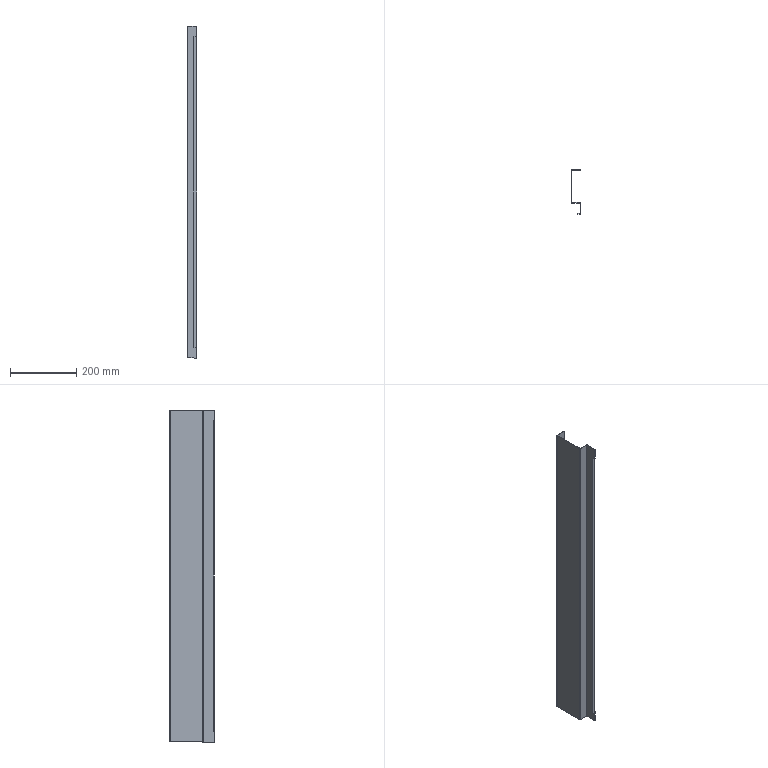Component | SolidWorks | SideUpperCrossbeam-2 | 1 solid | 58 faces | volume 293922 mm3 | plane 42 | cylinder 16 | commonest cylinder face diameters 11 x8 3.4 x4 0.4 x4